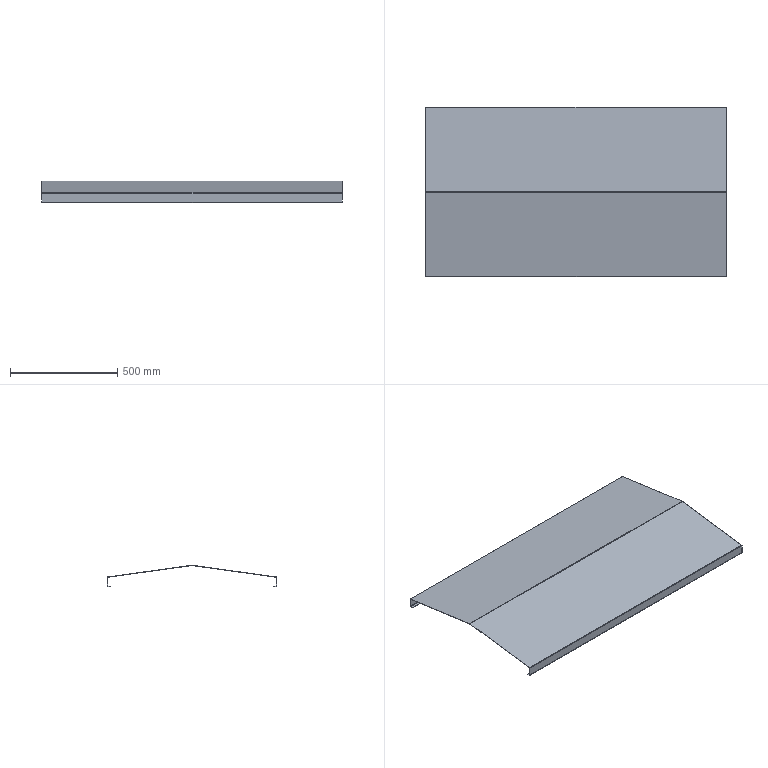Component | SolidWorks | TopCoverAssembly-1_TopCover-1 | 1 solid | 48 faces | volume 1907804 mm3 | plane 36 | cylinder 12 | commonest cylinder face diameters 6 x6 3 x6